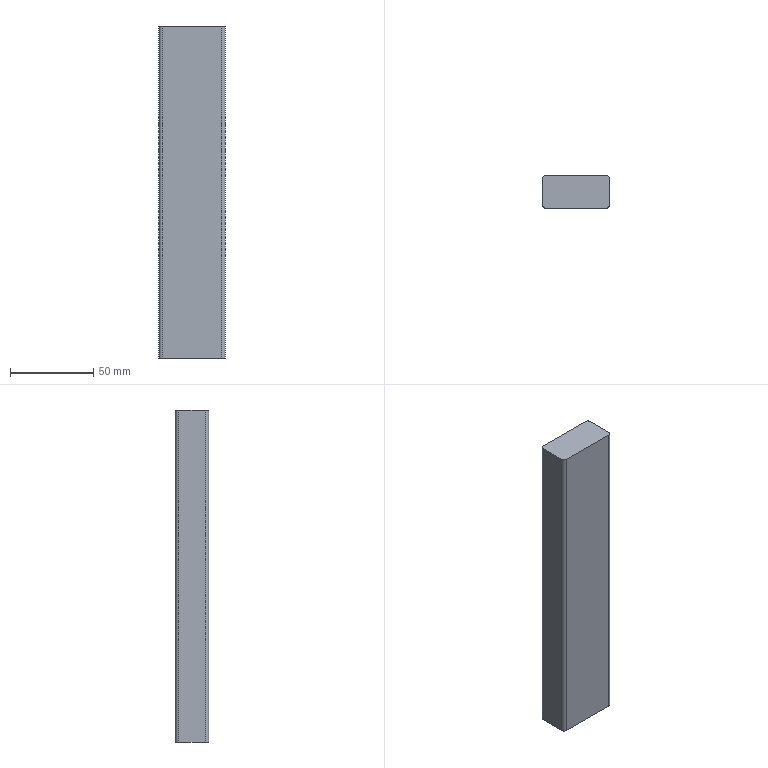Component | SolidWorks | Pillar-1 | 1 solid | 10 faces | box 40 x 20 x 200 mm | volume 159313 mm3 | plane 6 | cylinder 4 | commonest cylinder face diameters 4 x4 | material Aviation Aluminum-7075
build123d program:
from build123d import *

# Parameters (mm, degrees)
BOSS_EXTRUDE1_DEPTH = 200


with BuildPart() as part:
    # Sketch1 → Boss-Extrude1 (new body)
    with BuildSketch(Plane.XY):
        with BuildLine():
            Line((18, -10), (-18, -10))
            ThreePointArc((-18, -10), (-19.414, -9.414), (-20, -8))
            Line((-20, -8), (-20, 8))
            ThreePointArc((-20, 8), (-19.414, 9.414), (-18, 10))
            Line((-18, 10), (18, 10))
            ThreePointArc((18, 10), (19.414, 9.414), (20, 8))
            Line((20, 8), (20, -8))
            ThreePointArc((20, -8), (19.414, -9.414), (18, -10))
        make_face()
    extrude(amount=BOSS_EXTRUDE1_DEPTH)


solid = part.part

# Placed as in the assembly
solid = solid.moved(Location((-179.87, -416.626, 492.215), (0, 0, 0)))
STEP:
#1=COLOUR_RGB('',0.7922,0.8196,0.9333);
#2=FILL_AREA_STYLE_COLOUR('',#1);
#3=FILL_AREA_STYLE('',(#2));
#4=SURFACE_STYLE_FILL_AREA(#3);
#5=SURFACE_SIDE_STYLE('',(#4));
#6=SURFACE_STYLE_USAGE(.BOTH.,#5);
#7=PRESENTATION_STYLE_ASSIGNMENT((#6));
#8=CARTESIAN_POINT('',(-7.869,-16.088,27.253));
#9=VERTEX_POINT('',#8);
#10=CARTESIAN_POINT('',(-7.79,-16.009,27.253));
#11=VERTEX_POINT('',#10);
#12=CARTESIAN_POINT('',(-7.79,-16.088,27.253));
#13=DIRECTION('',(0.,0.,-1.));
#14=DIRECTION('',(-1.,0.,0.));
#15=AXIS2_PLACEMENT_3D('',#12,#13,#14);
#16=CIRCLE('',#15,0.07874);
#17=EDGE_CURVE('',#9,#11,#16,.T.);
#18=ORIENTED_EDGE('',*,*,#17,.T.);
#19=CARTESIAN_POINT('',(-7.79,-16.009,19.379));
#20=VERTEX_POINT('',#19);
#21=CARTESIAN_POINT('',(-7.79,-16.009,19.379));
#22=DIRECTION('',(-0.,-0.,1.));
#23=VECTOR('',#22,39.37);
#24=LINE('',#21,#23);
#25=EDGE_CURVE('',#20,#11,#24,.T.);
#26=ORIENTED_EDGE('',*,*,#25,.F.);
#27=CARTESIAN_POINT('',(-7.869,-16.088,19.379));
#28=VERTEX_POINT('',#27);
#29=CARTESIAN_POINT('',(-7.79,-16.088,19.379));
#30=DIRECTION('',(0.,0.,-1.));
#31=DIRECTION('',(-1.,0.,0.));
#32=AXIS2_PLACEMENT_3D('',#29,#30,#31);
#33=CIRCLE('',#32,0.07874);
#34=EDGE_CURVE('',#28,#20,#33,.T.);
#35=ORIENTED_EDGE('',*,*,#34,.F.);
#36=CARTESIAN_POINT('',(-7.869,-16.088,19.379));
#37=DIRECTION('',(-0.,-0.,1.));
#38=VECTOR('',#37,39.37);
#39=LINE('',#36,#38);
#40=EDGE_CURVE('',#28,#9,#39,.T.);
#41=ORIENTED_EDGE('',*,*,#40,.T.);
#42=EDGE_LOOP('',(#18,#26,#35,#41));
#43=FACE_OUTER_BOUND('',#42,.T.);
#44=CARTESIAN_POINT('',(-7.79,-16.088,19.379));
#45=DIRECTION('',(-0.,-0.,1.));
#46=DIRECTION('',(-1.,0.,0.));
#47=AXIS2_PLACEMENT_3D('',#44,#45,#46);
#48=CYLINDRICAL_SURFACE('',#47,0.07874);
#49=ADVANCED_FACE('',(#43),#48,.T.);
#50=CARTESIAN_POINT('',(-6.373,-16.009,27.253));
#51=VERTEX_POINT('',#50);
#52=CARTESIAN_POINT('',(-6.373,-16.009,27.253));
#53=DIRECTION('',(1.,-0.,0.));
#54=VECTOR('',#53,39.37);
#55=LINE('',#52,#54);
#56=EDGE_CURVE('',#11,#51,#55,.T.);
#57=ORIENTED_EDGE('',*,*,#56,.T.);
#58=CARTESIAN_POINT('',(-6.373,-16.009,19.379));
#59=VERTEX_POINT('',#58);
#60=CARTESIAN_POINT('',(-6.373,-16.009,19.379));
#61=DIRECTION('',(-0.,-0.,1.));
#62=VECTOR('',#61,39.37);
#63=LINE('',#60,#62);
#64=EDGE_CURVE('',#59,#51,#63,.T.);
#65=ORIENTED_EDGE('',*,*,#64,.F.);
#66=CARTESIAN_POINT('',(-6.373,-16.009,19.379));
#67=DIRECTION('',(1.,-0.,0.));
#68=VECTOR('',#67,39.37);
#69=LINE('',#66,#68);
#70=EDGE_CURVE('',#20,#59,#69,.T.);
#71=ORIENTED_EDGE('',*,*,#70,.F.);
#72=ORIENTED_EDGE('',*,*,#25,.T.);
#73=EDGE_LOOP('',(#57,#65,#71,#72));
#74=FACE_OUTER_BOUND('',#73,.T.);
#75=CARTESIAN_POINT('',(-6.373,-16.009,19.379));
#76=DIRECTION('',(-0.,-1.,-0.));
#77=DIRECTION('',(0.,0.,-1.));
#78=AXIS2_PLACEMENT_3D('',#75,#76,#77);
#79=PLANE('',#78);
#80=ADVANCED_FACE('',(#74),#79,.F.);
#81=CARTESIAN_POINT('',(-6.294,-16.088,27.253));
#82=VERTEX_POINT('',#81);
#83=CARTESIAN_POINT('',(-6.373,-16.088,27.253));
#84=DIRECTION('',(0.,0.,-1.));
#85=DIRECTION('',(1.,0.,0.));
#86=AXIS2_PLACEMENT_3D('',#83,#84,#85);
#87=CIRCLE('',#86,0.07874);
#88=EDGE_CURVE('',#51,#82,#87,.T.);
#89=ORIENTED_EDGE('',*,*,#88,.T.);
#90=CARTESIAN_POINT('',(-6.294,-16.088,19.379));
#91=VERTEX_POINT('',#90);
#92=CARTESIAN_POINT('',(-6.294,-16.088,19.379));
#93=DIRECTION('',(-0.,-0.,1.));
#94=VECTOR('',#93,39.37);
#95=LINE('',#92,#94);
#96=EDGE_CURVE('',#91,#82,#95,.T.);
#97=ORIENTED_EDGE('',*,*,#96,.F.);
#98=CARTESIAN_POINT('',(-6.373,-16.088,19.379));
#99=DIRECTION('',(0.,0.,-1.));
#100=DIRECTION('',(1.,0.,0.));
#101=AXIS2_PLACEMENT_3D('',#98,#99,#100);
#102=CIRCLE('',#101,0.07874);
#103=EDGE_CURVE('',#59,#91,#102,.T.);
#104=ORIENTED_EDGE('',*,*,#103,.F.);
#105=ORIENTED_EDGE('',*,*,#64,.T.);
#106=EDGE_LOOP('',(#89,#97,#104,#105));
#107=FACE_OUTER_BOUND('',#106,.T.);
#108=CARTESIAN_POINT('',(-6.373,-16.088,19.379));
#109=DIRECTION('',(-0.,-0.,1.));
#110=DIRECTION('',(-1.,0.,0.));
#111=AXIS2_PLACEMENT_3D('',#108,#109,#110);
#112=CYLINDRICAL_SURFACE('',#111,0.07874);
#113=ADVANCED_FACE('',(#107),#112,.T.);
#114=CARTESIAN_POINT('',(-6.294,-16.718,27.253));
#115=VERTEX_POINT('',#114);
#116=CARTESIAN_POINT('',(-6.294,-16.088,27.253));
#117=DIRECTION('',(-0.,-1.,-0.));
#118=VECTOR('',#117,39.37);
#119=LINE('',#116,#118);
#120=EDGE_CURVE('',#82,#115,#119,.T.);
#121=ORIENTED_EDGE('',*,*,#120,.T.);
#122=CARTESIAN_POINT('',(-6.294,-16.718,19.379));
#123=VERTEX_POINT('',#122);
#124=CARTESIAN_POINT('',(-6.294,-16.718,19.379));
#125=DIRECTION('',(-0.,-0.,1.));
#126=VECTOR('',#125,39.37);
#127=LINE('',#124,#126);
#128=EDGE_CURVE('',#123,#115,#127,.T.);
#129=ORIENTED_EDGE('',*,*,#128,.F.);
#130=CARTESIAN_POINT('',(-6.294,-16.088,19.379));
#131=DIRECTION('',(-0.,-1.,-0.));
#132=VECTOR('',#131,39.37);
#133=LINE('',#130,#132);
#134=EDGE_CURVE('',#91,#123,#133,.T.);
#135=ORIENTED_EDGE('',*,*,#134,.F.);
#136=ORIENTED_EDGE('',*,*,#96,.T.);
#137=EDGE_LOOP('',(#121,#129,#135,#136));
#138=FACE_OUTER_BOUND('',#137,.T.);
#139=CARTESIAN_POINT('',(-6.294,-16.088,19.379));
#140=DIRECTION('',(-1.,0.,-0.));
#141=DIRECTION('',(0.,0.,-1.));
#142=AXIS2_PLACEMENT_3D('',#139,#140,#141);
#143=PLANE('',#142);
#144=ADVANCED_FACE('',(#138),#143,.F.);
#145=CARTESIAN_POINT('',(-6.373,-16.796,27.253));
#146=VERTEX_POINT('',#145);
#147=CARTESIAN_POINT('',(-6.373,-16.718,27.253));
#148=DIRECTION('',(0.,0.,-1.));
#149=DIRECTION('',(1.,0.,0.));
#150=AXIS2_PLACEMENT_3D('',#147,#148,#149);
#151=CIRCLE('',#150,0.07874);
#152=EDGE_CURVE('',#115,#146,#151,.T.);
#153=ORIENTED_EDGE('',*,*,#152,.T.);
#154=CARTESIAN_POINT('',(-6.373,-16.796,19.379));
#155=VERTEX_POINT('',#154);
#156=CARTESIAN_POINT('',(-6.373,-16.796,19.379));
#157=DIRECTION('',(-0.,-0.,1.));
#158=VECTOR('',#157,39.37);
#159=LINE('',#156,#158);
#160=EDGE_CURVE('',#155,#146,#159,.T.);
#161=ORIENTED_EDGE('',*,*,#160,.F.);
#162=CARTESIAN_POINT('',(-6.373,-16.718,19.379));
#163=DIRECTION('',(0.,0.,-1.));
#164=DIRECTION('',(1.,0.,0.));
#165=AXIS2_PLACEMENT_3D('',#162,#163,#164);
#166=CIRCLE('',#165,0.07874);
#167=EDGE_CURVE('',#123,#155,#166,.T.);
#168=ORIENTED_EDGE('',*,*,#167,.F.);
#169=ORIENTED_EDGE('',*,*,#128,.T.);
#170=EDGE_LOOP('',(#153,#161,#168,#169));
#171=FACE_OUTER_BOUND('',#170,.T.);
#172=CARTESIAN_POINT('',(-6.373,-16.718,19.379));
#173=DIRECTION('',(-0.,-0.,1.));
#174=DIRECTION('',(-1.,0.,0.));
#175=AXIS2_PLACEMENT_3D('',#172,#173,#174);
#176=CYLINDRICAL_SURFACE('',#175,0.07874);
#177=ADVANCED_FACE('',(#171),#176,.T.);
#178=CARTESIAN_POINT('',(-7.79,-16.796,27.253));
#179=VERTEX_POINT('',#178);
#180=CARTESIAN_POINT('',(-6.373,-16.796,27.253));
#181=DIRECTION('',(-1.,0.,-0.));
#182=VECTOR('',#181,39.37);
#183=LINE('',#180,#182);
#184=EDGE_CURVE('',#146,#179,#183,.T.);
#185=ORIENTED_EDGE('',*,*,#184,.T.);
#186=CARTESIAN_POINT('',(-7.79,-16.796,19.379));
#187=VERTEX_POINT('',#186);
#188=CARTESIAN_POINT('',(-7.79,-16.796,19.379));
#189=DIRECTION('',(-0.,-0.,1.));
#190=VECTOR('',#189,39.37);
#191=LINE('',#188,#190);
#192=EDGE_CURVE('',#187,#179,#191,.T.);
#193=ORIENTED_EDGE('',*,*,#192,.F.);
#194=CARTESIAN_POINT('',(-6.373,-16.796,19.379));
#195=DIRECTION('',(-1.,0.,-0.));
#196=VECTOR('',#195,39.37);
#197=LINE('',#194,#196);
#198=EDGE_CURVE('',#155,#187,#197,.T.);
#199=ORIENTED_EDGE('',*,*,#198,.F.);
#200=ORIENTED_EDGE('',*,*,#160,.T.);
#201=EDGE_LOOP('',(#185,#193,#199,#200));
#202=FACE_OUTER_BOUND('',#201,.T.);
#203=CARTESIAN_POINT('',(-6.373,-16.796,19.379));
#204=DIRECTION('',(0.,1.,0.));
#205=DIRECTION('',(1.,-0.,0.));
#206=AXIS2_PLACEMENT_3D('',#203,#204,#205);
#207=PLANE('',#206);
#208=ADVANCED_FACE('',(#202),#207,.F.);
#209=CARTESIAN_POINT('',(-7.869,-16.718,27.253));
#210=VERTEX_POINT('',#209);
#211=CARTESIAN_POINT('',(-7.79,-16.718,27.253));
#212=DIRECTION('',(0.,0.,-1.));
#213=DIRECTION('',(1.,0.,0.));
#214=AXIS2_PLACEMENT_3D('',#211,#212,#213);
#215=CIRCLE('',#214,0.07874);
#216=EDGE_CURVE('',#179,#210,#215,.T.);
#217=ORIENTED_EDGE('',*,*,#216,.T.);
#218=CARTESIAN_POINT('',(-7.869,-16.718,19.379));
#219=VERTEX_POINT('',#218);
#220=CARTESIAN_POINT('',(-7.869,-16.718,19.379));
#221=DIRECTION('',(-0.,-0.,1.));
#222=VECTOR('',#221,39.37);
#223=LINE('',#220,#222);
#224=EDGE_CURVE('',#219,#210,#223,.T.);
#225=ORIENTED_EDGE('',*,*,#224,.F.);
#226=CARTESIAN_POINT('',(-7.79,-16.718,19.379));
#227=DIRECTION('',(0.,0.,-1.));
#228=DIRECTION('',(1.,0.,0.));
#229=AXIS2_PLACEMENT_3D('',#226,#227,#228);
#230=CIRCLE('',#229,0.07874);
#231=EDGE_CURVE('',#187,#219,#230,.T.);
#232=ORIENTED_EDGE('',*,*,#231,.F.);
#233=ORIENTED_EDGE('',*,*,#192,.T.);
#234=EDGE_LOOP('',(#217,#225,#232,#233));
#235=FACE_OUTER_BOUND('',#234,.T.);
#236=CARTESIAN_POINT('',(-7.79,-16.718,19.379));
#237=DIRECTION('',(-0.,-0.,1.));
#238=DIRECTION('',(-1.,0.,0.));
#239=AXIS2_PLACEMENT_3D('',#236,#237,#238);
#240=CYLINDRICAL_SURFACE('',#239,0.07874);
#241=ADVANCED_FACE('',(#235),#240,.T.);
#242=CARTESIAN_POINT('',(-7.869,-16.088,27.253));
#243=DIRECTION('',(0.,1.,0.));
#244=VECTOR('',#243,39.37);
#245=LINE('',#242,#244);
#246=EDGE_CURVE('',#210,#9,#245,.T.);
#247=ORIENTED_EDGE('',*,*,#246,.T.);
#248=ORIENTED_EDGE('',*,*,#40,.F.);
#249=CARTESIAN_POINT('',(-7.869,-16.088,19.379));
#250=DIRECTION('',(0.,1.,0.));
#251=VECTOR('',#250,39.37);
#252=LINE('',#249,#251);
#253=EDGE_CURVE('',#219,#28,#252,.T.);
#254=ORIENTED_EDGE('',*,*,#253,.F.);
#255=ORIENTED_EDGE('',*,*,#224,.T.);
#256=EDGE_LOOP('',(#247,#248,#254,#255));
#257=FACE_OUTER_BOUND('',#256,.T.);
#258=CARTESIAN_POINT('',(-7.869,-16.088,19.379));
#259=DIRECTION('',(1.,-0.,0.));
#260=DIRECTION('',(-0.,-0.,1.));
#261=AXIS2_PLACEMENT_3D('',#258,#259,#260);
#262=PLANE('',#261);
#263=ADVANCED_FACE('',(#257),#262,.F.);
#264=ORIENTED_EDGE('',*,*,#34,.T.);
#265=ORIENTED_EDGE('',*,*,#70,.T.);
#266=ORIENTED_EDGE('',*,*,#103,.T.);
#267=ORIENTED_EDGE('',*,*,#134,.T.);
#268=ORIENTED_EDGE('',*,*,#167,.T.);
#269=ORIENTED_EDGE('',*,*,#198,.T.);
#270=ORIENTED_EDGE('',*,*,#231,.T.);
#271=ORIENTED_EDGE('',*,*,#253,.T.);
#272=EDGE_LOOP('',(#264,#265,#266,#267,#268,#269,#270,#271));
#273=FACE_OUTER_BOUND('',#272,.T.);
#274=CARTESIAN_POINT('',(-7.79,-16.088,19.379));
#275=DIRECTION('',(-0.,-0.,1.));
#276=DIRECTION('',(-1.,0.,-0.));
#277=AXIS2_PLACEMENT_3D('',#274,#275,#276);
#278=PLANE('',#277);
#279=ADVANCED_FACE('',(#273),#278,.F.);
#280=ORIENTED_EDGE('',*,*,#17,.F.);
#281=ORIENTED_EDGE('',*,*,#246,.F.);
#282=ORIENTED_EDGE('',*,*,#216,.F.);
#283=ORIENTED_EDGE('',*,*,#184,.F.);
#284=ORIENTED_EDGE('',*,*,#152,.F.);
#285=ORIENTED_EDGE('',*,*,#120,.F.);
#286=ORIENTED_EDGE('',*,*,#88,.F.);
#287=ORIENTED_EDGE('',*,*,#56,.F.);
#288=EDGE_LOOP('',(#280,#281,#282,#283,#284,#285,#286,#287));
#289=FACE_OUTER_BOUND('',#288,.T.);
#290=CARTESIAN_POINT('',(-7.79,-16.088,27.253));
#291=DIRECTION('',(-0.,-0.,1.));
#292=DIRECTION('',(-1.,0.,-0.));
#293=AXIS2_PLACEMENT_3D('',#290,#291,#292);
#294=PLANE('',#293);
#295=ADVANCED_FACE('',(#289),#294,.T.);
#296=CLOSED_SHELL('',(#49,#80,#113,#144,#177,#208,#241,#263,#279,#295));
#297=MANIFOLD_SOLID_BREP('',#296);
#298=STYLED_ITEM('',(#7),#297);
#299=PRESENTATION_LAYER_ASSIGNMENT('','',(#298));
#300=CARTESIAN_POINT('',(0.,0.,0.));
#301=DIRECTION('',(0.,0.,1.));
#302=DIRECTION('',(1.,0.,0.));
#303=AXIS2_PLACEMENT_3D('',#300,#301,#302);
#304=(LENGTH_UNIT()NAMED_UNIT(*)SI_UNIT($,.METRE.));
#305=LENGTH_MEASURE_WITH_UNIT(LENGTH_MEASURE(0.0254),#304);
#306=DIMENSIONAL_EXPONENTS(1.,0.,0.,0.,0.,0.,0.);
#307=(CONVERSION_BASED_UNIT('',#305)LENGTH_UNIT()NAMED_UNIT(#306));
#308=UNCERTAINTY_MEASURE_WITH_UNIT(LENGTH_MEASURE(0.00001),#307,'','');
#309=(NAMED_UNIT(*)PLANE_ANGLE_UNIT()SI_UNIT($,.RADIAN.));
#310=(NAMED_UNIT(*)SI_UNIT($,.STERADIAN.)SOLID_ANGLE_UNIT());
#311=(GEOMETRIC_REPRESENTATION_CONTEXT(3)GLOBAL_UNCERTAINTY_ASSIGNED_CONTEXT((#308))GLOBAL_UNIT_ASSIGNED_CONTEXT((#307,#309,#310))REPRESENTATION_CONTEXT('',''));
#312=ADVANCED_BREP_SHAPE_REPRESENTATION('',(#297,#303),#311);
#313=(LENGTH_UNIT()NAMED_UNIT(*)SI_UNIT($,.METRE.));
#314=LENGTH_MEASURE_WITH_UNIT(LENGTH_MEASURE(0.0254),#313);
#315=DIMENSIONAL_EXPONENTS(1.,0.,0.,0.,0.,0.,0.);
#316=(CONVERSION_BASED_UNIT('',#314)LENGTH_UNIT()NAMED_UNIT(#315));
#317=UNCERTAINTY_MEASURE_WITH_UNIT(LENGTH_MEASURE(0.00001),#316,'','');
#318=(NAMED_UNIT(*)PLANE_ANGLE_UNIT()SI_UNIT($,.RADIAN.));
#319=(NAMED_UNIT(*)SI_UNIT($,.STERADIAN.)SOLID_ANGLE_UNIT());
#320=(GEOMETRIC_REPRESENTATION_CONTEXT(3)GLOBAL_UNCERTAINTY_ASSIGNED_CONTEXT((#317))GLOBAL_UNIT_ASSIGNED_CONTEXT((#316,#318,#319))REPRESENTATION_CONTEXT('',''));
#321=MECHANICAL_DESIGN_GEOMETRIC_PRESENTATION_REPRESENTATION('',(#298),#320);